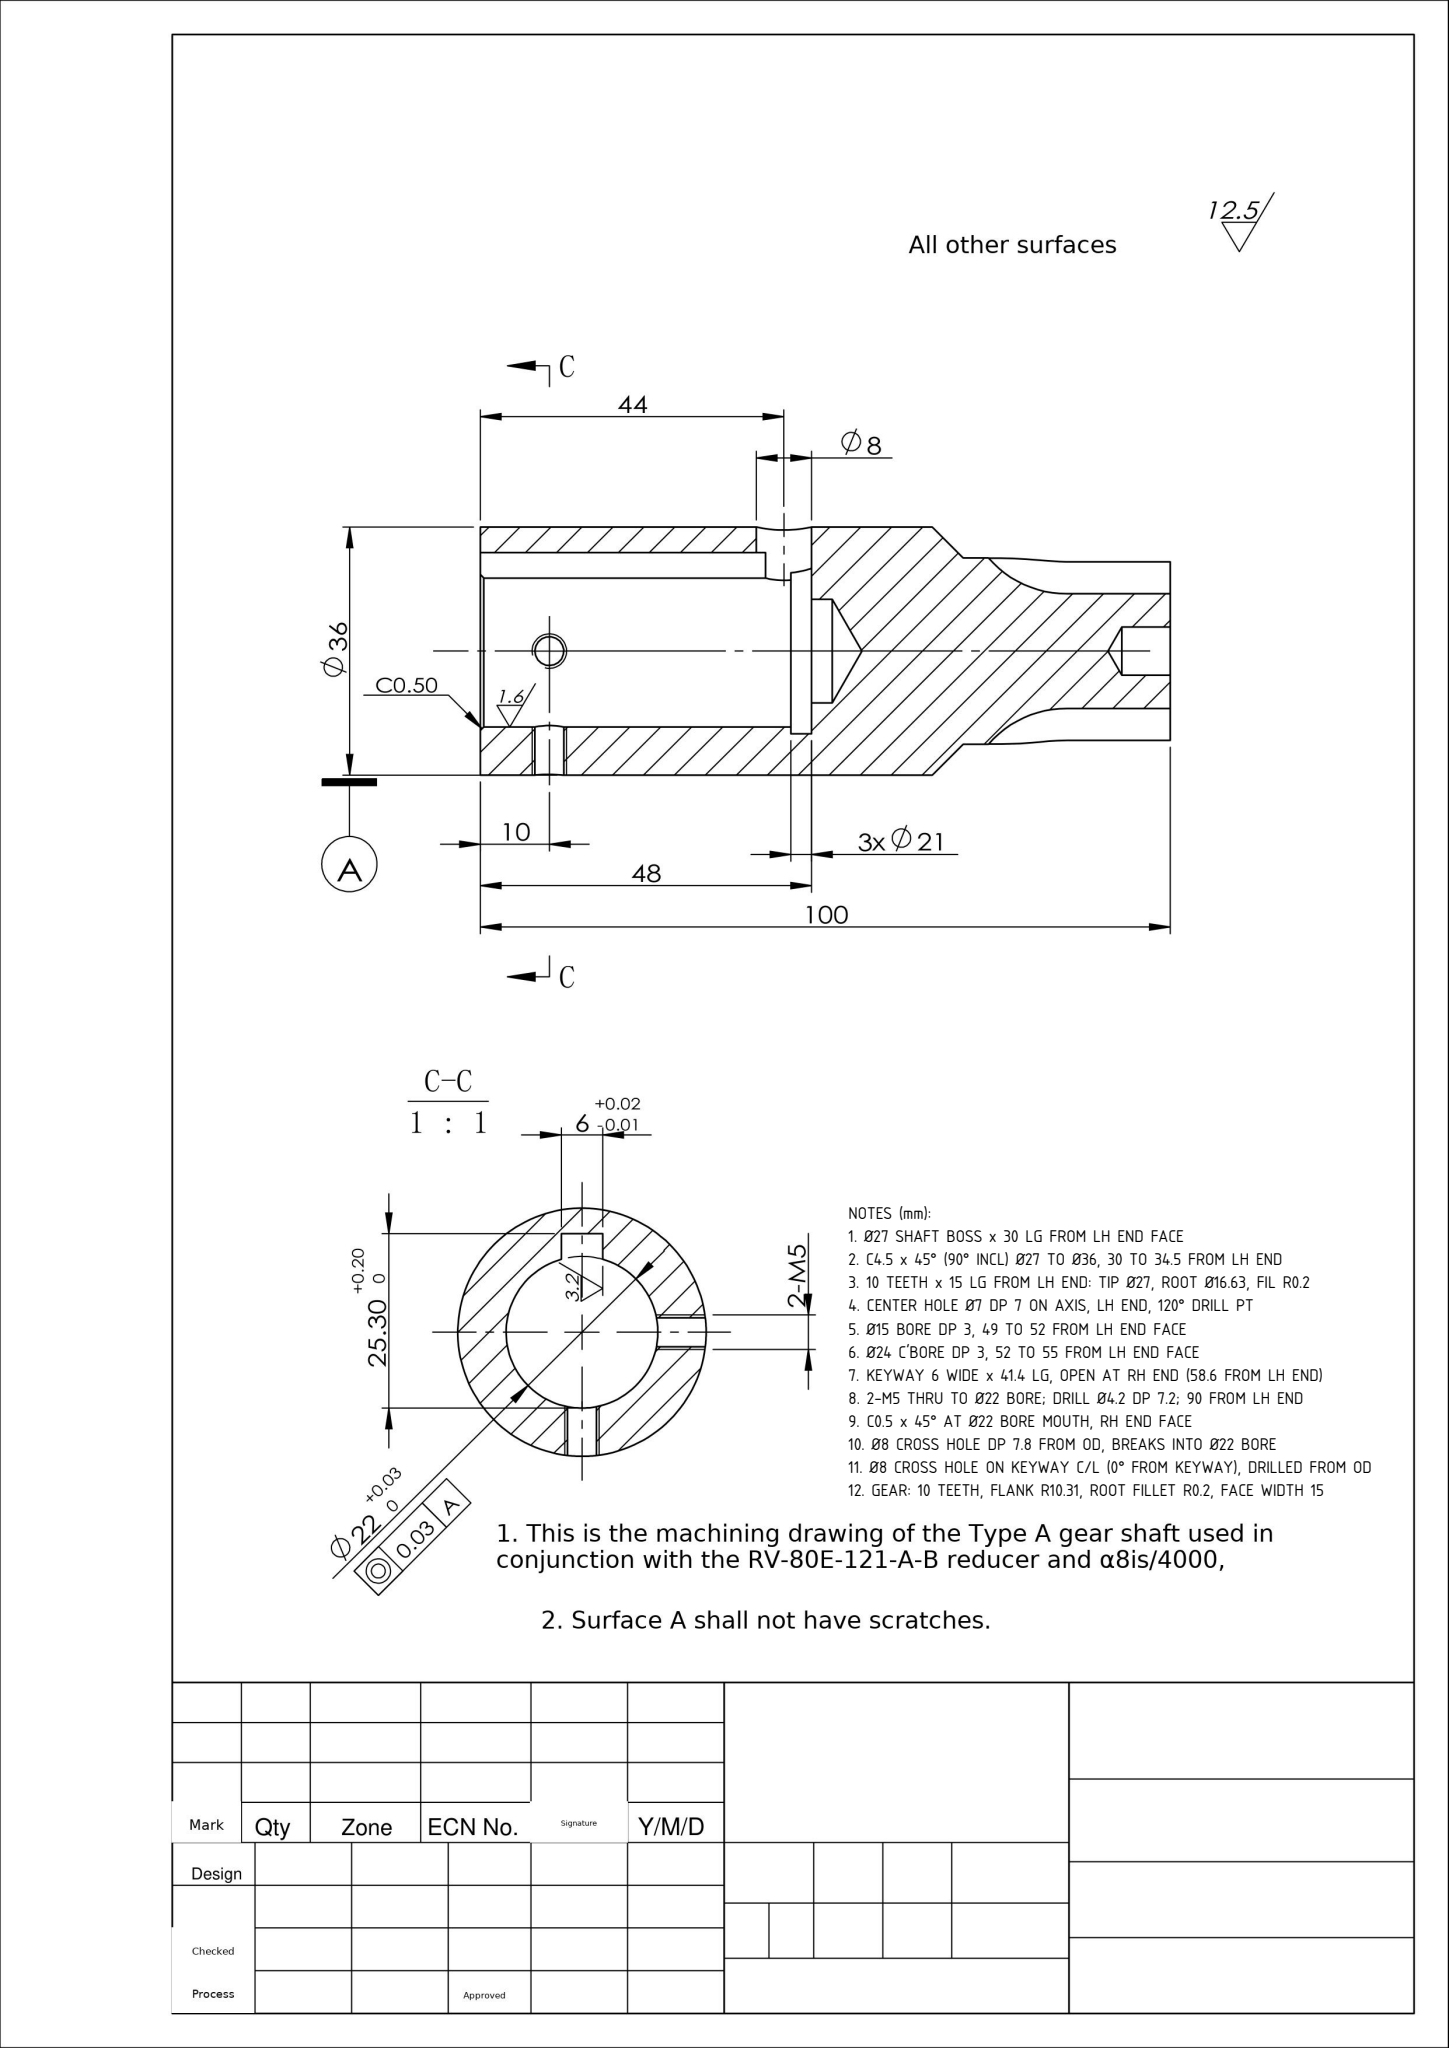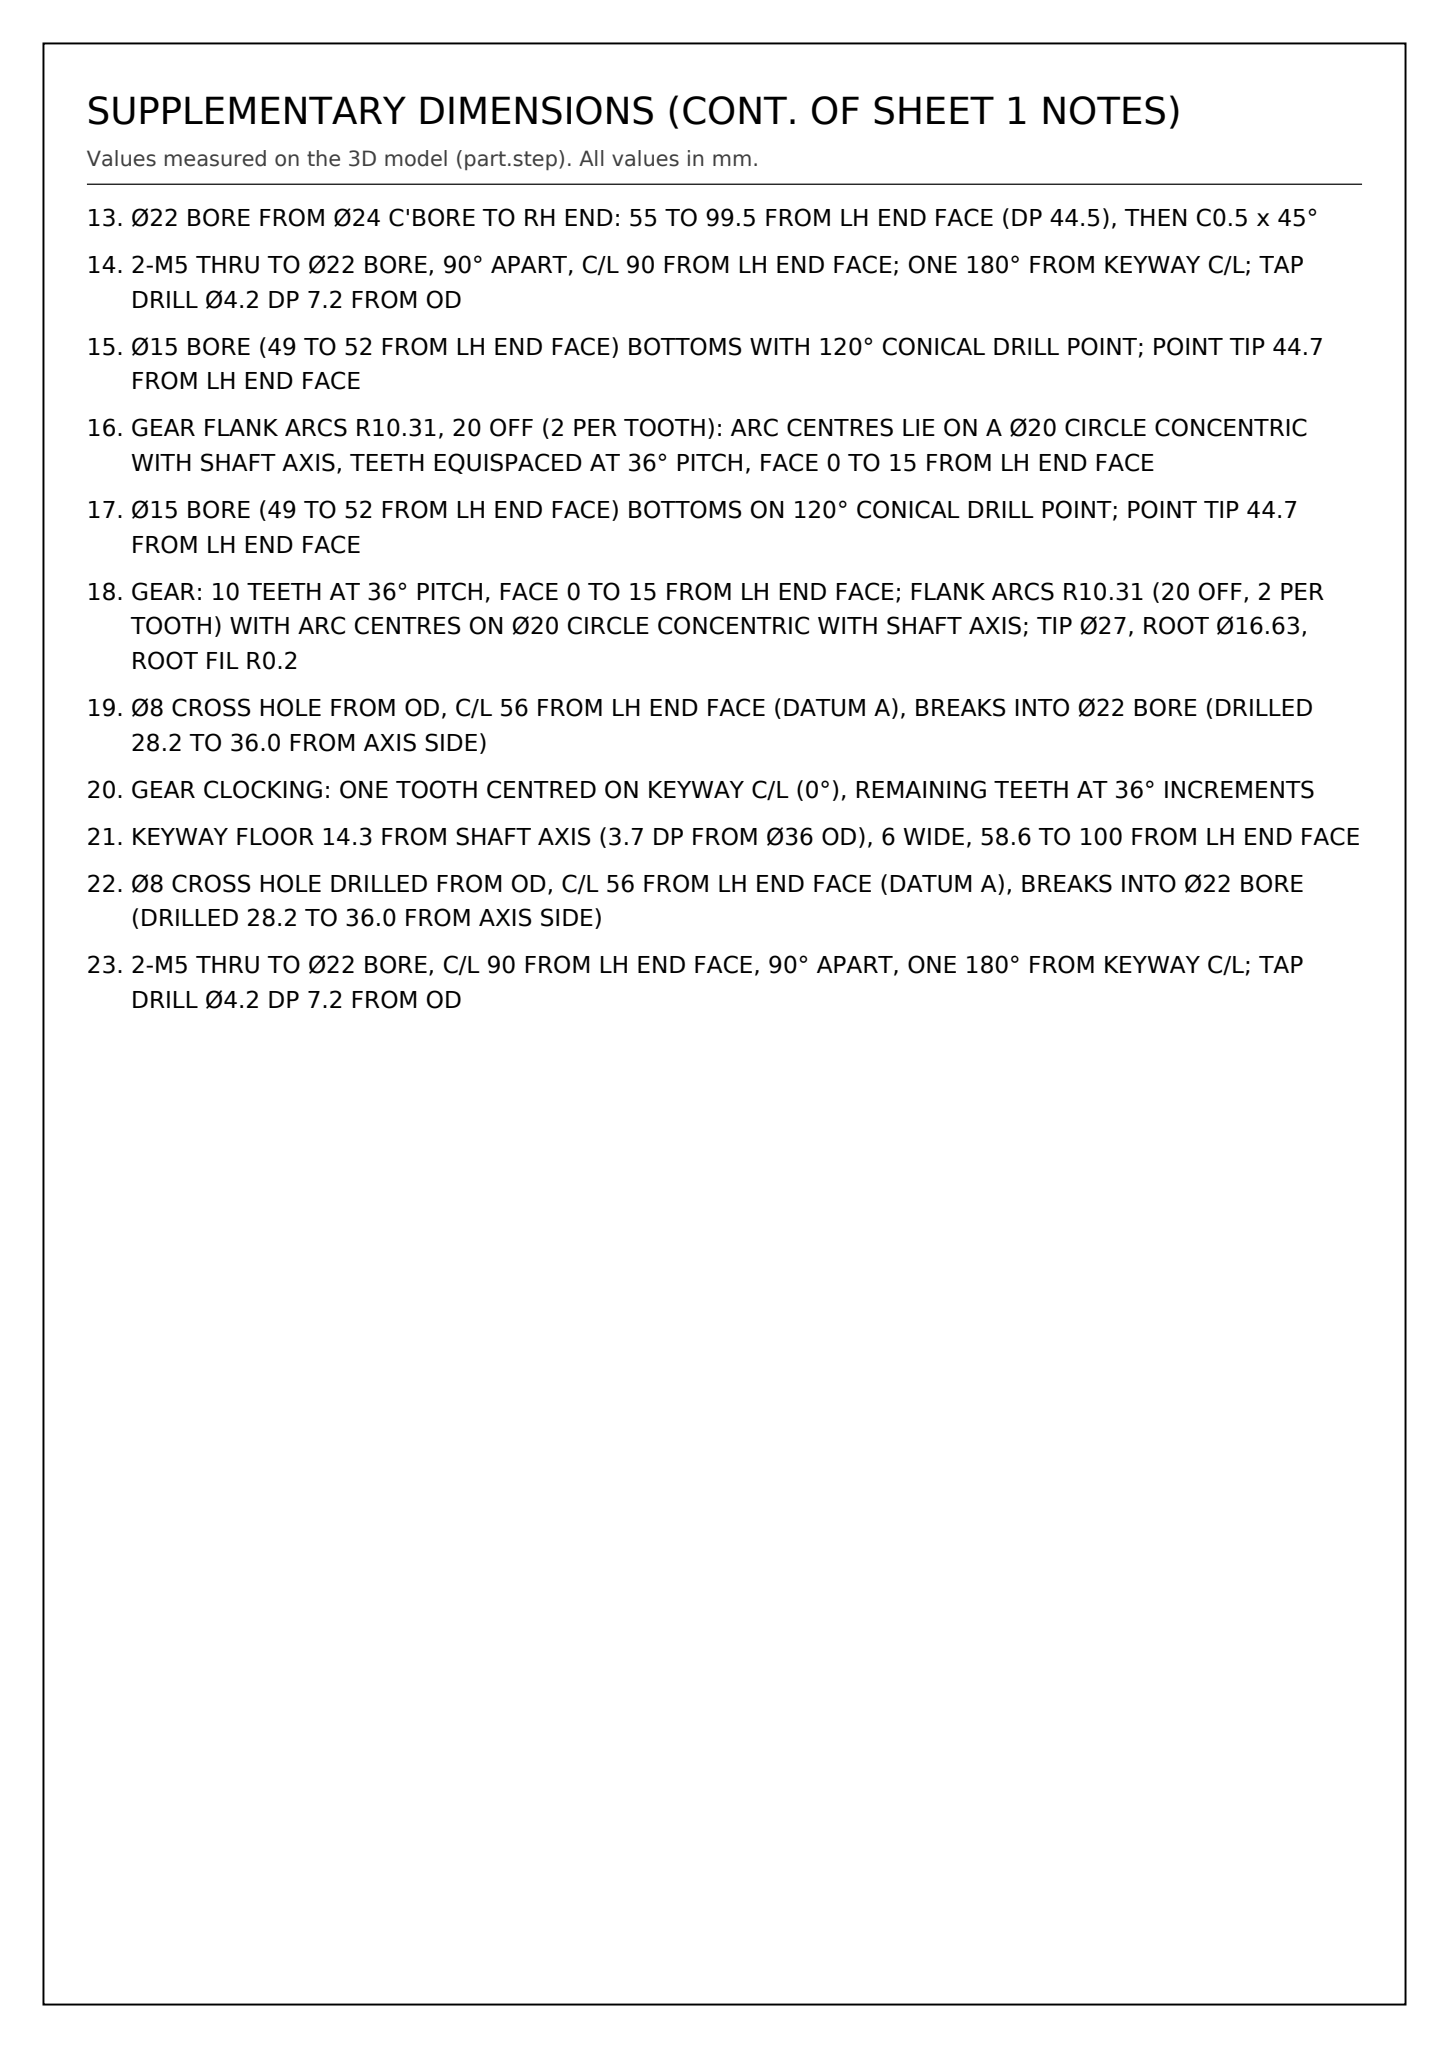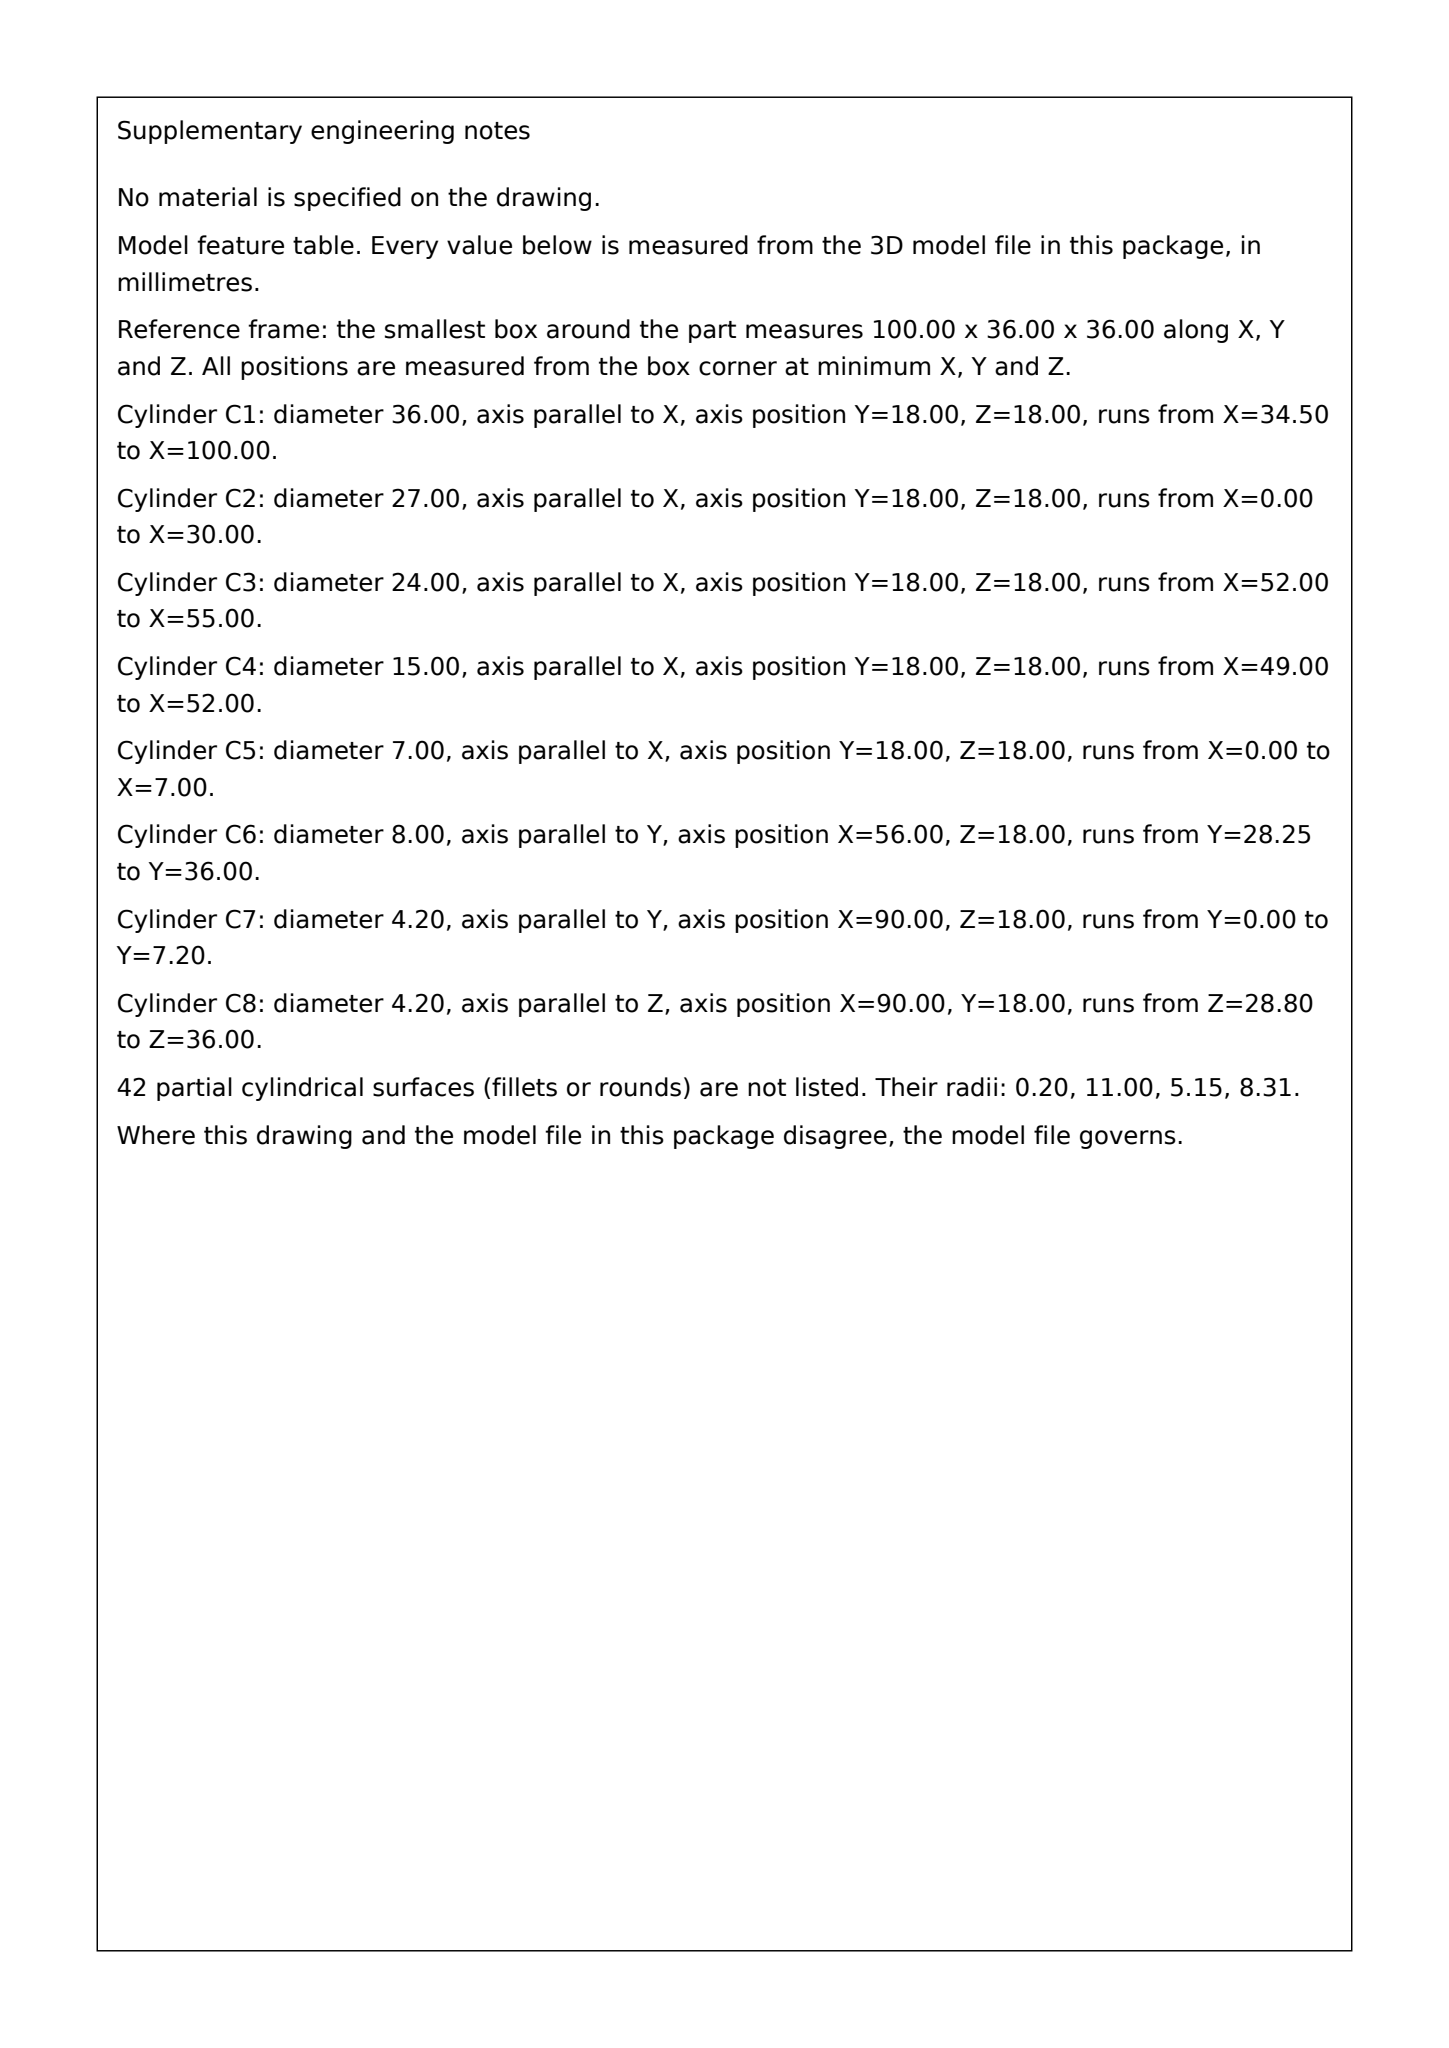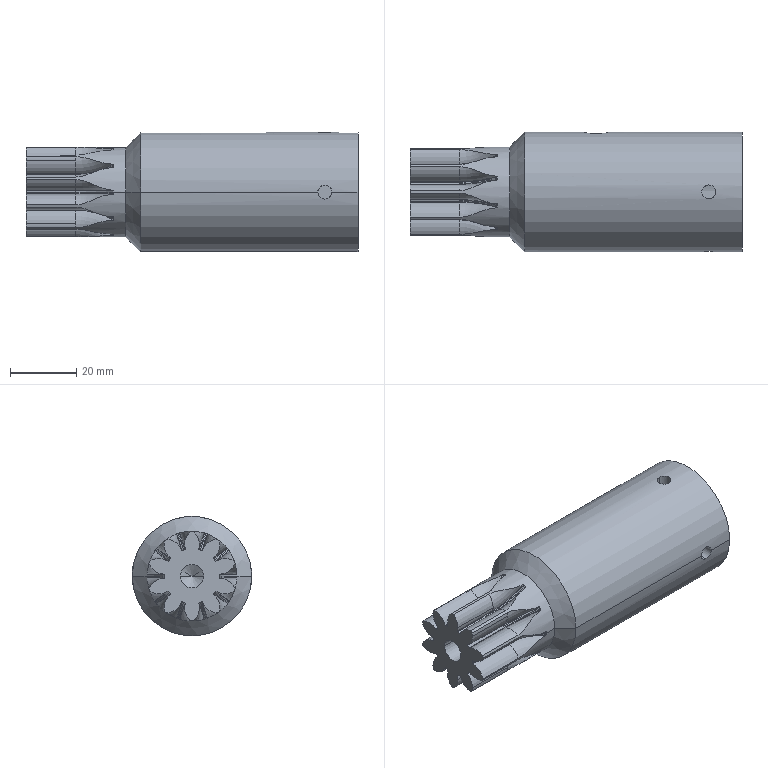Part | SolidWorks | mm | 1 solid | 172 faces | box 100 x 36 x 36 mm | volume 62930 mm3 | cylinder 78 | torus 60 | spline 20 | cone 7 | plane 7 | commonest cylinder face diameters 0.4 x26 10.308 x24 16.625 x11 4.2 x4 8 x2 36 x2 27 x2 7 x2
Drawing notes:
Ø27 SHAFT BOSS x 30 LG FROM LH END FACE | from the solid: cylinder boss/shaft dia 27, axis x, from 0.0 to 30.0
C4.5 x 45° (90° INCL) Ø27 TO Ø36, 30 TO 34.5 FROM LH END | from the solid: cone 90 deg, ref_dia 36, bbox_from x=30.0, size 4.5; Ø36 shaft starts x=34.5
10 TEETH x 15 LG FROM LH END: TIP Ø27, ROOT Ø16.63, FIL R0.2 | from the solid: 20 flank arcs R5.155 + 20 root arcs R0.2 in 10 pairs at 36° pitch, x 0-15; root circle arc dia 16.63; end face extent 27 across
CENTER HOLE Ø7 DP 7 ON AXIS, LH END, 120° DRILL PT | from the solid: hole/bore dia 7.0 axis x from 0.0 to 7.0; cone 120 deg ref_dia 7.0 bbox_from x=7.0
Ø15 BORE DP 3, 49 TO 52 FROM LH END FACE | from the solid: hole/bore dia 15.0 axis x from 49.0 to 52.0; plane x=52
Ø24 C'BORE DP 3, 52 TO 55 FROM LH END FACE | from the solid: hole/bore dia 24.0 axis x from 52.0 to 55.0; planes x=52, x=55
KEYWAY 6 WIDE x 41.4 LG, OPEN AT RH END (58.6 FROM LH END) | from the solid: keyway planes y=32.3 and z=15/21 extent x 58.6-100.0, width z 15-21
2-M5 THRU TO Ø22 BORE; DRILL Ø4.2 DP 7.2; 90 FROM LH END | from the solid: hole dia 4.2 axis y at x=90 from 0-7.2 and dia 4.2 axis z at x=90 from 28.8-36.0
C0.5 x 45° AT Ø22 BORE MOUTH, RH END FACE | from the solid: cone 90 deg ref_dia 22.0 bbox_from x=99.5, size 0.5; Ø22 bore ends x=99.5
Ø8 CROSS HOLE DP 7.8 FROM OD, BREAKS INTO Ø22 BORE | from the solid: hole/bore dia 8.0 axis y at x=56, z=18, from y=28.2 to 36.0 (OD); Ø22 bore r=11 > 10.2
Ø8 CROSS HOLE ON KEYWAY C/L (0° FROM KEYWAY), DRILLED FROM OD | from the solid: Ø8 axis along +y from y=36 to 28.2; keyway top face y=32.3 also on +y side -> same angular position
GEAR: 10 TEETH, FLANK R10.31, ROOT FILLET R0.2, FACE WIDTH 15 | from the solid: 20 convex R10.31 arcs (2/tooth) + R0.2 fillets, x=0 to 15; tip Ø27, root Ø16.63
Ø22 BORE FROM Ø24 C'BORE TO RH END: 55 TO 99.5 FROM LH END FACE (DP 44.5), THEN C0.5 x 45° | from the solid: cylinders: hole/bore Ø22.0 on x axis from 55.0 to 99.5; cone 90° ref dia 22.0 at x 99.5-100.0
2-M5 THRU TO Ø22 BORE, 90° APART, C/L 90 FROM LH END FACE; ONE 180° FROM KEYWAY C/L; TAP DRILL Ø4.2 DP 7.2 FROM OD | from the solid: cylinders: hole/bore Ø4.2 on y axis at x=90.0, z=18.0, 0.0 to 7.2; hole/bore Ø4.2 on z axis at x=90.0, y=18.0, 28.8 to 36.0
Ø15 BORE (49 TO 52 FROM LH END FACE) BOTTOMS WITH 120° CONICAL DRILL POINT; POINT TIP 44.7 FROM LH END FACE | from the solid: hole/bore Ø15 on x axis from 49.0 to 52.0 plus cones 120° with bbox_from x=44.7 (height 4.3) on the Ø15 bore axis (y,z = 18,18)
GEAR FLANK ARCS R10.31, 20 OFF (2 PER TOOTH): ARC CENTRES LIE ON A Ø20 CIRCLE CONCENTRIC WITH SHAFT AXIS, TEETH EQUISPACED AT 36° PITCH, FACE 0 TO 15 FROM LH END FACE | from the solid: 20 convex arcs R10.31, axis x, from 0.0 to 15.0, centres (y,z) e.g. (10.0,12.0), (14.8,27.5), (26.0,24.0) all at radius 10.0 from shaft axis (18,18)
Ø15 BORE (49 TO 52 FROM LH END FACE) BOTTOMS ON 120° CONICAL DRILL POINT; POINT TIP 44.7 FROM LH END FACE | from the solid: cones[included_angle 120.0, bbox_from x=44.7] together with hole/bore Ø15 x-axis from 49.0 to 52.0
GEAR: 10 TEETH AT 36° PITCH, FACE 0 TO 15 FROM LH END FACE; FLANK ARCS R10.31 (20 OFF, 2 PER TOOTH) WITH ARC CENTRES ON Ø20 CIRCLE CONCENTRIC WITH SHAFT AXIS; TIP Ø27, ROOT Ø16.63, ROOT FIL R0.2 | from the solid: convex arc (round/outer radius) 10.31 x-axis, 20 instances at centres offset 10.0 from axis (18.0,18.0), from 0.0 to 15.0; convex arc 16.63 root; boss/shaft Ø27 from 0.0 to 30.0
Ø8 CROSS HOLE FROM OD, C/L 56 FROM LH END FACE (DATUM A), BREAKS INTO Ø22 BORE (DRILLED 28.2 TO 36.0 FROM AXIS SIDE) | from the solid: cylinders: hole/bore Ø8.0, axis y at x=56.0, z=18.0, from 28.2 to 36.0
GEAR CLOCKING: ONE TOOTH CENTRED ON KEYWAY C/L (0°), REMAINING TEETH AT 36° INCREMENTS | from the solid: convex arc R10.31 centres at (y,z)=(28.0,17.8) and (28.0,18.2) straddle z=18 on +y side, same side as keyway (planes z=15/z=21, floor y=32.3)
KEYWAY FLOOR 14.3 FROM SHAFT AXIS (3.7 DP FROM Ø36 OD), 6 WIDE, 58.6 TO 100 FROM LH END FACE | from the solid: axis_planes: y=32.3 over x 58.6-100, z 15.0-21.0; z=15 and z=21 side faces; Ø36 OD cylinder
Ø8 CROSS HOLE DRILLED FROM OD, C/L 56 FROM LH END FACE (DATUM A), BREAKS INTO Ø22 BORE (DRILLED 28.2 TO 36.0 FROM AXIS SIDE) | from the solid: cylinders: hole/bore Ø8.0, axis y, axis_pos x=56.0 z=18.0, from 28.2 to 36.0
2-M5 THRU TO Ø22 BORE, C/L 90 FROM LH END FACE, 90° APART, ONE 180° FROM KEYWAY C/L; TAP DRILL Ø4.2 DP 7.2 FROM OD | from the solid: cylinders: hole/bore Ø4.2 axis y at x=90.0, from 0.0 to 7.2 and hole/bore Ø4.2 axis z at x=90.0, from 28.8 to 36.0